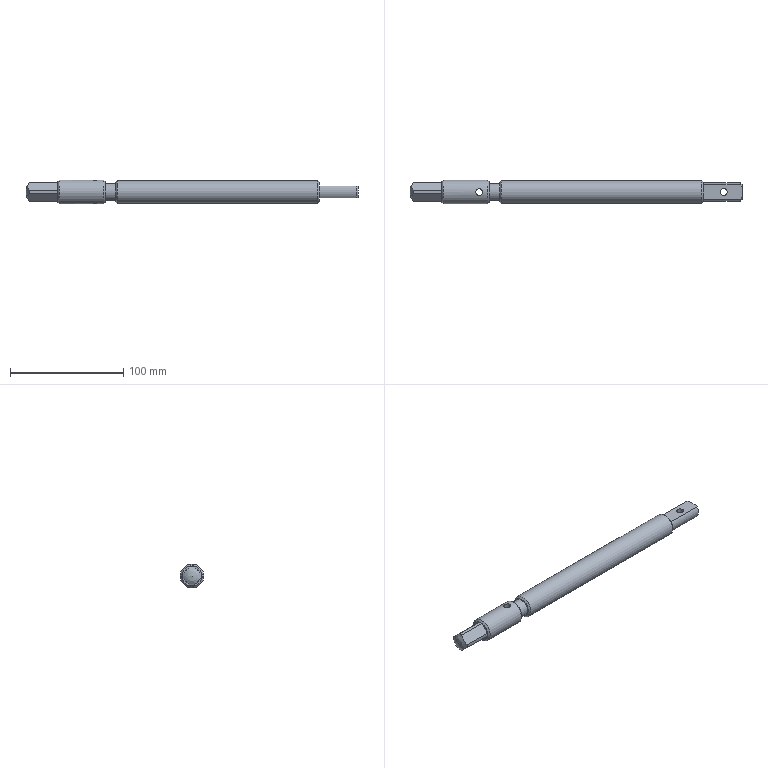Component | NX | HORIZONTALLEADSCREW | 1 solid | 29 faces | volume 81606 mm3 | cylinder 11 | plane 11 | cone 6 | sphere 1 | commonest cylinder face diameters 17 x4 16 x2 6 x2 21 x1 20 x1 15 x1